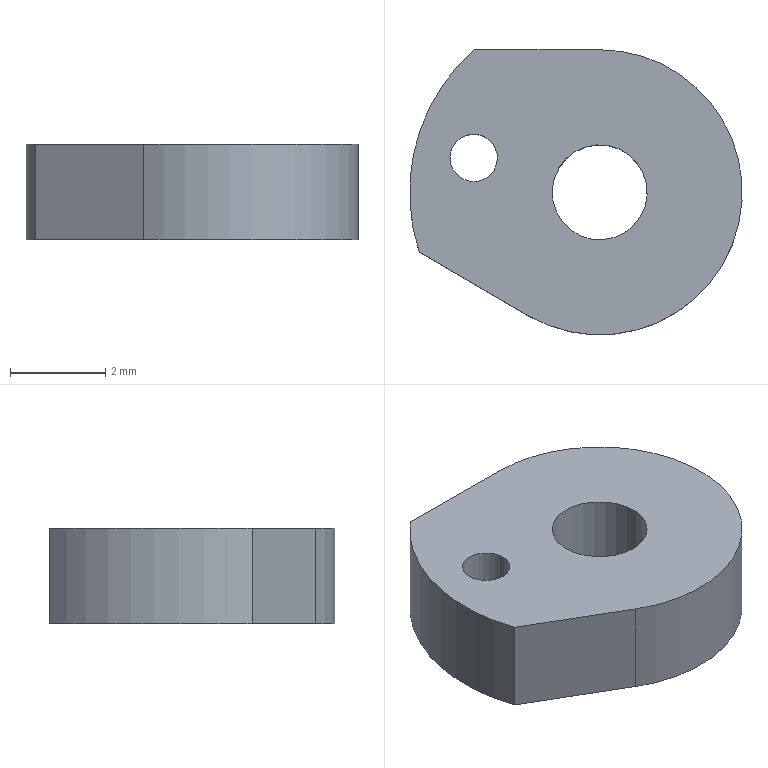Component | SolidWorks | DeflectionCam(Rear)-2 | 1 solid | 11 faces | box 7 x 6.01 x 2 mm | volume 60 mm3 | cylinder 7 | plane 4 | commonest cylinder face diameters 1 x2 2 x2 6 x2 8 x1
build123d program:
from build123d import *

# Parameters (mm, degrees)
SKETCH1_R           = 1
BOSS_EXTRUDE1_DEPTH = 2
SKETCH2_R           = 0.5
CUT_EXTRUDE1_DEPTH  = 2


with BuildPart() as part:
    # Sketch1 → Boss-Extrude1 (new body)
    with BuildSketch(Plane.XY):
        with BuildLine():
            Line((-5.155, 2.996), (-7.798, 2.859))
            ThreePointArc((-7.798, 2.859), (-8.912, 0.8339), (-8.72, -1.47))
            Line((-8.72, -1.47), (-6.363, -2.672))
            ThreePointArc((-6.363, -2.672), (-2.066, -0.6254), (-5.155, 2.996))
        make_face()
        with Locations((-5, 0)):
            Circle(SKETCH1_R, mode=Mode.SUBTRACT)
    extrude(amount=-BOSS_EXTRUDE1_DEPTH)

    # Sketch2 → Cut-Extrude1 (cut)
    with BuildSketch(Plane.XY):
        with Locations((-7.69, 0.5733)):
            Circle(SKETCH2_R)
    extrude(amount=-CUT_EXTRUDE1_DEPTH, mode=Mode.SUBTRACT)


solid = part.part

# Placed as in the assembly
solid = solid.moved(Location((17.492, -3.781, 7), (0, 0, -3.225)))
STEP:
#1=COLOUR_RGB('',0.7922,0.8196,0.9333);
#2=FILL_AREA_STYLE_COLOUR('',#1);
#3=FILL_AREA_STYLE('',(#2));
#4=SURFACE_STYLE_FILL_AREA(#3);
#5=SURFACE_SIDE_STYLE('',(#4));
#6=SURFACE_STYLE_USAGE(.BOTH.,#5);
#7=PRESENTATION_STYLE_ASSIGNMENT((#6));
#8=CARTESIAN_POINT('',(0.368,-0.1082,0.1969));
#9=VERTEX_POINT('',#8);
#10=CARTESIAN_POINT('',(0.4073,-0.1104,0.1969));
#11=VERTEX_POINT('',#10);
#12=CARTESIAN_POINT('',(0.3877,-0.1093,0.1969));
#13=DIRECTION('',(-0.,-0.,1.));
#14=DIRECTION('',(0.9984,-0.05626,0.));
#15=AXIS2_PLACEMENT_3D('',#12,#13,#14);
#16=CIRCLE('',#15,0.01969);
#17=EDGE_CURVE('',#9,#11,#16,.T.);
#18=ORIENTED_EDGE('',*,*,#17,.F.);
#19=CARTESIAN_POINT('',(0.368,-0.1082,0.2756));
#20=VERTEX_POINT('',#19);
#21=CARTESIAN_POINT('',(0.368,-0.1082,0.1969));
#22=DIRECTION('',(-0.,-0.,1.));
#23=VECTOR('',#22,39.37);
#24=LINE('',#21,#23);
#25=EDGE_CURVE('',#9,#20,#24,.T.);
#26=ORIENTED_EDGE('',*,*,#25,.T.);
#27=CARTESIAN_POINT('',(0.4073,-0.1104,0.2756));
#28=VERTEX_POINT('',#27);
#29=CARTESIAN_POINT('',(0.3877,-0.1093,0.2756));
#30=DIRECTION('',(-0.,-0.,1.));
#31=DIRECTION('',(0.9984,-0.05626,0.));
#32=AXIS2_PLACEMENT_3D('',#29,#30,#31);
#33=CIRCLE('',#32,0.01969);
#34=EDGE_CURVE('',#20,#28,#33,.T.);
#35=ORIENTED_EDGE('',*,*,#34,.T.);
#36=CARTESIAN_POINT('',(0.4073,-0.1104,0.1969));
#37=DIRECTION('',(-0.,-0.,1.));
#38=VECTOR('',#37,39.37);
#39=LINE('',#36,#38);
#40=EDGE_CURVE('',#11,#28,#39,.T.);
#41=ORIENTED_EDGE('',*,*,#40,.F.);
#42=EDGE_LOOP('',(#18,#26,#35,#41));
#43=FACE_OUTER_BOUND('',#42,.T.);
#44=CARTESIAN_POINT('',(0.3877,-0.1093,0.1969));
#45=DIRECTION('',(-0.,-0.,1.));
#46=DIRECTION('',(0.9984,-0.05626,0.));
#47=AXIS2_PLACEMENT_3D('',#44,#45,#46);
#48=CYLINDRICAL_SURFACE('',#47,0.01969);
#49=ADVANCED_FACE('',(#43),#48,.F.);
#50=CARTESIAN_POINT('',(0.4528,-0.1356,0.1969));
#51=VERTEX_POINT('',#50);
#52=CARTESIAN_POINT('',(0.5314,-0.14,0.1969));
#53=VERTEX_POINT('',#52);
#54=CARTESIAN_POINT('',(0.4921,-0.1378,0.1969));
#55=DIRECTION('',(-0.,-0.,1.));
#56=DIRECTION('',(0.9984,-0.05626,0.));
#57=AXIS2_PLACEMENT_3D('',#54,#55,#56);
#58=CIRCLE('',#57,0.03937);
#59=EDGE_CURVE('',#51,#53,#58,.T.);
#60=ORIENTED_EDGE('',*,*,#59,.F.);
#61=CARTESIAN_POINT('',(0.4528,-0.1356,0.2756));
#62=VERTEX_POINT('',#61);
#63=CARTESIAN_POINT('',(0.4528,-0.1356,0.1969));
#64=DIRECTION('',(-0.,-0.,1.));
#65=VECTOR('',#64,39.37);
#66=LINE('',#63,#65);
#67=EDGE_CURVE('',#51,#62,#66,.T.);
#68=ORIENTED_EDGE('',*,*,#67,.T.);
#69=CARTESIAN_POINT('',(0.5314,-0.14,0.2756));
#70=VERTEX_POINT('',#69);
#71=CARTESIAN_POINT('',(0.4921,-0.1378,0.2756));
#72=DIRECTION('',(-0.,-0.,1.));
#73=DIRECTION('',(0.9984,-0.05626,0.));
#74=AXIS2_PLACEMENT_3D('',#71,#72,#73);
#75=CIRCLE('',#74,0.03937);
#76=EDGE_CURVE('',#62,#70,#75,.T.);
#77=ORIENTED_EDGE('',*,*,#76,.T.);
#78=CARTESIAN_POINT('',(0.5314,-0.14,0.1969));
#79=DIRECTION('',(-0.,-0.,1.));
#80=VECTOR('',#79,39.37);
#81=LINE('',#78,#80);
#82=EDGE_CURVE('',#53,#70,#81,.T.);
#83=ORIENTED_EDGE('',*,*,#82,.F.);
#84=EDGE_LOOP('',(#60,#68,#77,#83));
#85=FACE_OUTER_BOUND('',#84,.T.);
#86=CARTESIAN_POINT('',(0.4921,-0.1378,0.1969));
#87=DIRECTION('',(-0.,-0.,1.));
#88=DIRECTION('',(0.9984,-0.05626,0.));
#89=AXIS2_PLACEMENT_3D('',#86,#87,#88);
#90=CYLINDRICAL_SURFACE('',#89,0.03937);
#91=ADVANCED_FACE('',(#85),#90,.F.);
#92=CARTESIAN_POINT('',(0.4326,-0.2398,0.1969));
#93=VERTEX_POINT('',#92);
#94=CARTESIAN_POINT('',(0.61,-0.1444,0.1969));
#95=VERTEX_POINT('',#94);
#96=CARTESIAN_POINT('',(0.4921,-0.1378,0.1969));
#97=DIRECTION('',(-0.,-0.,1.));
#98=DIRECTION('',(0.9984,-0.05626,0.));
#99=AXIS2_PLACEMENT_3D('',#96,#97,#98);
#100=CIRCLE('',#99,0.1181);
#101=EDGE_CURVE('',#93,#95,#100,.T.);
#102=ORIENTED_EDGE('',*,*,#101,.T.);
#103=CARTESIAN_POINT('',(0.61,-0.1444,0.2756));
#104=VERTEX_POINT('',#103);
#105=CARTESIAN_POINT('',(0.61,-0.1444,0.1969));
#106=DIRECTION('',(-0.,-0.,1.));
#107=VECTOR('',#106,39.37);
#108=LINE('',#105,#107);
#109=EDGE_CURVE('',#95,#104,#108,.T.);
#110=ORIENTED_EDGE('',*,*,#109,.T.);
#111=CARTESIAN_POINT('',(0.4326,-0.2398,0.2756));
#112=VERTEX_POINT('',#111);
#113=CARTESIAN_POINT('',(0.4921,-0.1378,0.2756));
#114=DIRECTION('',(-0.,-0.,1.));
#115=DIRECTION('',(0.9984,-0.05626,0.));
#116=AXIS2_PLACEMENT_3D('',#113,#114,#115);
#117=CIRCLE('',#116,0.1181);
#118=EDGE_CURVE('',#112,#104,#117,.T.);
#119=ORIENTED_EDGE('',*,*,#118,.F.);
#120=CARTESIAN_POINT('',(0.4326,-0.2398,0.1969));
#121=DIRECTION('',(-0.,-0.,1.));
#122=VECTOR('',#121,39.37);
#123=LINE('',#120,#122);
#124=EDGE_CURVE('',#93,#112,#123,.T.);
#125=ORIENTED_EDGE('',*,*,#124,.F.);
#126=EDGE_LOOP('',(#102,#110,#119,#125));
#127=FACE_OUTER_BOUND('',#126,.T.);
#128=CARTESIAN_POINT('',(0.4921,-0.1378,0.1969));
#129=DIRECTION('',(-0.,-0.,1.));
#130=DIRECTION('',(0.9984,-0.05626,0.));
#131=AXIS2_PLACEMENT_3D('',#128,#129,#130);
#132=CYLINDRICAL_SURFACE('',#131,0.1181);
#133=ADVANCED_FACE('',(#127),#132,.T.);
#134=ORIENTED_EDGE('',*,*,#109,.F.);
#135=CARTESIAN_POINT('',(0.4927,-0.01969,0.1969));
#136=VERTEX_POINT('',#135);
#137=CARTESIAN_POINT('',(0.4921,-0.1378,0.1969));
#138=DIRECTION('',(-0.,-0.,1.));
#139=DIRECTION('',(0.9984,-0.05626,0.));
#140=AXIS2_PLACEMENT_3D('',#137,#138,#139);
#141=CIRCLE('',#140,0.1181);
#142=EDGE_CURVE('',#95,#136,#141,.T.);
#143=ORIENTED_EDGE('',*,*,#142,.T.);
#144=CARTESIAN_POINT('',(0.4927,-0.01969,0.2756));
#145=VERTEX_POINT('',#144);
#146=CARTESIAN_POINT('',(0.4927,-0.01969,0.1969));
#147=DIRECTION('',(-0.,-0.,1.));
#148=VECTOR('',#147,39.37);
#149=LINE('',#146,#148);
#150=EDGE_CURVE('',#136,#145,#149,.T.);
#151=ORIENTED_EDGE('',*,*,#150,.T.);
#152=CARTESIAN_POINT('',(0.4921,-0.1378,0.2756));
#153=DIRECTION('',(-0.,-0.,1.));
#154=DIRECTION('',(0.9984,-0.05626,0.));
#155=AXIS2_PLACEMENT_3D('',#152,#153,#154);
#156=CIRCLE('',#155,0.1181);
#157=EDGE_CURVE('',#104,#145,#156,.T.);
#158=ORIENTED_EDGE('',*,*,#157,.F.);
#159=EDGE_LOOP('',(#134,#143,#151,#158));
#160=FACE_OUTER_BOUND('',#159,.T.);
#161=CARTESIAN_POINT('',(0.4921,-0.1378,0.1969));
#162=DIRECTION('',(-0.,-0.,1.));
#163=DIRECTION('',(0.9984,-0.05626,0.));
#164=AXIS2_PLACEMENT_3D('',#161,#162,#163);
#165=CYLINDRICAL_SURFACE('',#164,0.1181);
#166=ADVANCED_FACE('',(#160),#165,.T.);
#167=CARTESIAN_POINT('',(0.3426,-0.1873,0.2756));
#168=VERTEX_POINT('',#167);
#169=CARTESIAN_POINT('',(0.4326,-0.2398,0.2756));
#170=DIRECTION('',(0.8638,-0.5039,0.));
#171=VECTOR('',#170,39.37);
#172=LINE('',#169,#171);
#173=EDGE_CURVE('',#168,#112,#172,.T.);
#174=ORIENTED_EDGE('',*,*,#173,.F.);
#175=CARTESIAN_POINT('',(0.3426,-0.1873,0.1969));
#176=VERTEX_POINT('',#175);
#177=CARTESIAN_POINT('',(0.3426,-0.1873,0.1969));
#178=DIRECTION('',(-0.,-0.,1.));
#179=VECTOR('',#178,39.37);
#180=LINE('',#177,#179);
#181=EDGE_CURVE('',#176,#168,#180,.T.);
#182=ORIENTED_EDGE('',*,*,#181,.F.);
#183=CARTESIAN_POINT('',(0.4326,-0.2398,0.1969));
#184=DIRECTION('',(0.8638,-0.5039,0.));
#185=VECTOR('',#184,39.37);
#186=LINE('',#183,#185);
#187=EDGE_CURVE('',#176,#93,#186,.T.);
#188=ORIENTED_EDGE('',*,*,#187,.T.);
#189=ORIENTED_EDGE('',*,*,#124,.T.);
#190=EDGE_LOOP('',(#174,#182,#188,#189));
#191=FACE_OUTER_BOUND('',#190,.T.);
#192=CARTESIAN_POINT('',(0.4326,-0.2398,0.1969));
#193=DIRECTION('',(-0.5039,-0.8638,0.));
#194=DIRECTION('',(0.8638,-0.5039,0.));
#195=AXIS2_PLACEMENT_3D('',#192,#193,#194);
#196=PLANE('',#195);
#197=ADVANCED_FACE('',(#191),#196,.T.);
#198=CARTESIAN_POINT('',(0.3885,-0.01922,0.2756));
#199=VERTEX_POINT('',#198);
#200=CARTESIAN_POINT('',(0.4921,-0.1378,0.2756));
#201=DIRECTION('',(-0.,-0.,1.));
#202=DIRECTION('',(0.9984,-0.05626,0.));
#203=AXIS2_PLACEMENT_3D('',#200,#201,#202);
#204=CIRCLE('',#203,0.1575);
#205=EDGE_CURVE('',#199,#168,#204,.T.);
#206=ORIENTED_EDGE('',*,*,#205,.F.);
#207=CARTESIAN_POINT('',(0.3885,-0.01922,0.1969));
#208=VERTEX_POINT('',#207);
#209=CARTESIAN_POINT('',(0.3885,-0.01922,0.1969));
#210=DIRECTION('',(-0.,-0.,1.));
#211=VECTOR('',#210,39.37);
#212=LINE('',#209,#211);
#213=EDGE_CURVE('',#208,#199,#212,.T.);
#214=ORIENTED_EDGE('',*,*,#213,.F.);
#215=CARTESIAN_POINT('',(0.4921,-0.1378,0.1969));
#216=DIRECTION('',(-0.,-0.,1.));
#217=DIRECTION('',(0.9984,-0.05626,0.));
#218=AXIS2_PLACEMENT_3D('',#215,#216,#217);
#219=CIRCLE('',#218,0.1575);
#220=EDGE_CURVE('',#208,#176,#219,.T.);
#221=ORIENTED_EDGE('',*,*,#220,.T.);
#222=ORIENTED_EDGE('',*,*,#181,.T.);
#223=EDGE_LOOP('',(#206,#214,#221,#222));
#224=FACE_OUTER_BOUND('',#223,.T.);
#225=CARTESIAN_POINT('',(0.4921,-0.1378,0.1969));
#226=DIRECTION('',(-0.,-0.,1.));
#227=DIRECTION('',(0.9984,-0.05626,0.));
#228=AXIS2_PLACEMENT_3D('',#225,#226,#227);
#229=CYLINDRICAL_SURFACE('',#228,0.1575);
#230=ADVANCED_FACE('',(#224),#229,.T.);
#231=CARTESIAN_POINT('',(0.4927,-0.01969,0.2756));
#232=DIRECTION('',(-1.,0.004495,0.));
#233=VECTOR('',#232,39.37);
#234=LINE('',#231,#233);
#235=EDGE_CURVE('',#145,#199,#234,.T.);
#236=ORIENTED_EDGE('',*,*,#235,.F.);
#237=ORIENTED_EDGE('',*,*,#150,.F.);
#238=CARTESIAN_POINT('',(0.4927,-0.01969,0.1969));
#239=DIRECTION('',(-1.,0.004495,0.));
#240=VECTOR('',#239,39.37);
#241=LINE('',#238,#240);
#242=EDGE_CURVE('',#136,#208,#241,.T.);
#243=ORIENTED_EDGE('',*,*,#242,.T.);
#244=ORIENTED_EDGE('',*,*,#213,.T.);
#245=EDGE_LOOP('',(#236,#237,#243,#244));
#246=FACE_OUTER_BOUND('',#245,.T.);
#247=CARTESIAN_POINT('',(0.4927,-0.01969,0.1969));
#248=DIRECTION('',(0.004495,1.,-0.));
#249=DIRECTION('',(-1.,0.004495,0.));
#250=AXIS2_PLACEMENT_3D('',#247,#248,#249);
#251=PLANE('',#250);
#252=ADVANCED_FACE('',(#246),#251,.T.);
#253=CARTESIAN_POINT('',(0.3877,-0.1093,0.1969));
#254=DIRECTION('',(-0.,-0.,1.));
#255=DIRECTION('',(0.9984,-0.05626,0.));
#256=AXIS2_PLACEMENT_3D('',#253,#254,#255);
#257=CIRCLE('',#256,0.01969);
#258=EDGE_CURVE('',#11,#9,#257,.T.);
#259=ORIENTED_EDGE('',*,*,#258,.T.);
#260=ORIENTED_EDGE('',*,*,#17,.T.);
#261=EDGE_LOOP('',(#259,#260));
#262=FACE_BOUND('',#261,.T.);
#263=CARTESIAN_POINT('',(0.4921,-0.1378,0.1969));
#264=DIRECTION('',(-0.,-0.,1.));
#265=DIRECTION('',(0.9984,-0.05626,0.));
#266=AXIS2_PLACEMENT_3D('',#263,#264,#265);
#267=CIRCLE('',#266,0.03937);
#268=EDGE_CURVE('',#53,#51,#267,.T.);
#269=ORIENTED_EDGE('',*,*,#268,.T.);
#270=ORIENTED_EDGE('',*,*,#59,.T.);
#271=EDGE_LOOP('',(#269,#270));
#272=FACE_BOUND('',#271,.T.);
#273=ORIENTED_EDGE('',*,*,#101,.F.);
#274=ORIENTED_EDGE('',*,*,#187,.F.);
#275=ORIENTED_EDGE('',*,*,#220,.F.);
#276=ORIENTED_EDGE('',*,*,#242,.F.);
#277=ORIENTED_EDGE('',*,*,#142,.F.);
#278=EDGE_LOOP('',(#273,#274,#275,#276,#277));
#279=FACE_OUTER_BOUND('',#278,.T.);
#280=CARTESIAN_POINT('',(0.4921,-0.1378,0.1969));
#281=DIRECTION('',(0.,-0.,1.));
#282=DIRECTION('',(0.9984,-0.05626,-0.));
#283=AXIS2_PLACEMENT_3D('',#280,#281,#282);
#284=PLANE('',#283);
#285=ADVANCED_FACE('',(#262,#272,#279),#284,.F.);
#286=CARTESIAN_POINT('',(0.3877,-0.1093,0.2756));
#287=DIRECTION('',(-0.,-0.,1.));
#288=DIRECTION('',(0.9984,-0.05626,0.));
#289=AXIS2_PLACEMENT_3D('',#286,#287,#288);
#290=CIRCLE('',#289,0.01969);
#291=EDGE_CURVE('',#28,#20,#290,.T.);
#292=ORIENTED_EDGE('',*,*,#291,.F.);
#293=ORIENTED_EDGE('',*,*,#34,.F.);
#294=EDGE_LOOP('',(#292,#293));
#295=FACE_BOUND('',#294,.T.);
#296=CARTESIAN_POINT('',(0.4921,-0.1378,0.2756));
#297=DIRECTION('',(-0.,-0.,1.));
#298=DIRECTION('',(0.9984,-0.05626,0.));
#299=AXIS2_PLACEMENT_3D('',#296,#297,#298);
#300=CIRCLE('',#299,0.03937);
#301=EDGE_CURVE('',#70,#62,#300,.T.);
#302=ORIENTED_EDGE('',*,*,#301,.F.);
#303=ORIENTED_EDGE('',*,*,#76,.F.);
#304=EDGE_LOOP('',(#302,#303));
#305=FACE_BOUND('',#304,.T.);
#306=ORIENTED_EDGE('',*,*,#118,.T.);
#307=ORIENTED_EDGE('',*,*,#157,.T.);
#308=ORIENTED_EDGE('',*,*,#235,.T.);
#309=ORIENTED_EDGE('',*,*,#205,.T.);
#310=ORIENTED_EDGE('',*,*,#173,.T.);
#311=EDGE_LOOP('',(#306,#307,#308,#309,#310));
#312=FACE_OUTER_BOUND('',#311,.T.);
#313=CARTESIAN_POINT('',(0.4921,-0.1378,0.2756));
#314=DIRECTION('',(0.,-0.,1.));
#315=DIRECTION('',(0.9984,-0.05626,-0.));
#316=AXIS2_PLACEMENT_3D('',#313,#314,#315);
#317=PLANE('',#316);
#318=ADVANCED_FACE('',(#295,#305,#312),#317,.T.);
#319=ORIENTED_EDGE('',*,*,#67,.F.);
#320=ORIENTED_EDGE('',*,*,#268,.F.);
#321=ORIENTED_EDGE('',*,*,#82,.T.);
#322=ORIENTED_EDGE('',*,*,#301,.T.);
#323=EDGE_LOOP('',(#319,#320,#321,#322));
#324=FACE_OUTER_BOUND('',#323,.T.);
#325=CARTESIAN_POINT('',(0.4921,-0.1378,0.1969));
#326=DIRECTION('',(-0.,-0.,1.));
#327=DIRECTION('',(0.9984,-0.05626,0.));
#328=AXIS2_PLACEMENT_3D('',#325,#326,#327);
#329=CYLINDRICAL_SURFACE('',#328,0.03937);
#330=ADVANCED_FACE('',(#324),#329,.F.);
#331=ORIENTED_EDGE('',*,*,#25,.F.);
#332=ORIENTED_EDGE('',*,*,#258,.F.);
#333=ORIENTED_EDGE('',*,*,#40,.T.);
#334=ORIENTED_EDGE('',*,*,#291,.T.);
#335=EDGE_LOOP('',(#331,#332,#333,#334));
#336=FACE_OUTER_BOUND('',#335,.T.);
#337=CARTESIAN_POINT('',(0.3877,-0.1093,0.1969));
#338=DIRECTION('',(-0.,-0.,1.));
#339=DIRECTION('',(0.9984,-0.05626,0.));
#340=AXIS2_PLACEMENT_3D('',#337,#338,#339);
#341=CYLINDRICAL_SURFACE('',#340,0.01969);
#342=ADVANCED_FACE('',(#336),#341,.F.);
#343=CLOSED_SHELL('',(#49,#91,#133,#166,#197,#230,#252,#285,#318,#330,#342));
#344=MANIFOLD_SOLID_BREP('',#343);
#345=STYLED_ITEM('',(#7),#344);
#346=(LENGTH_UNIT()NAMED_UNIT(*)SI_UNIT($,.METRE.));
#347=LENGTH_MEASURE_WITH_UNIT(LENGTH_MEASURE(0.0254),#346);
#348=DIMENSIONAL_EXPONENTS(1.,0.,0.,0.,0.,0.,0.);
#349=(CONVERSION_BASED_UNIT('',#347)LENGTH_UNIT()NAMED_UNIT(#348));
#350=UNCERTAINTY_MEASURE_WITH_UNIT(LENGTH_MEASURE(0.00001),#349,'','');
#351=(NAMED_UNIT(*)PLANE_ANGLE_UNIT()SI_UNIT($,.RADIAN.));
#352=(NAMED_UNIT(*)SI_UNIT($,.STERADIAN.)SOLID_ANGLE_UNIT());
#353=(GEOMETRIC_REPRESENTATION_CONTEXT(3)GLOBAL_UNCERTAINTY_ASSIGNED_CONTEXT((#350))GLOBAL_UNIT_ASSIGNED_CONTEXT((#349,#351,#352))REPRESENTATION_CONTEXT('',''));
#354=MECHANICAL_DESIGN_GEOMETRIC_PRESENTATION_REPRESENTATION('',(#345),#353);
#355=CARTESIAN_POINT('',(0.,0.,0.));
#356=DIRECTION('',(0.,0.,1.));
#357=DIRECTION('',(1.,0.,0.));
#358=AXIS2_PLACEMENT_3D('',#355,#356,#357);
#359=(LENGTH_UNIT()NAMED_UNIT(*)SI_UNIT($,.METRE.));
#360=LENGTH_MEASURE_WITH_UNIT(LENGTH_MEASURE(0.0254),#359);
#361=DIMENSIONAL_EXPONENTS(1.,0.,0.,0.,0.,0.,0.);
#362=(CONVERSION_BASED_UNIT('',#360)LENGTH_UNIT()NAMED_UNIT(#361));
#363=UNCERTAINTY_MEASURE_WITH_UNIT(LENGTH_MEASURE(0.00001),#362,'','');
#364=(NAMED_UNIT(*)PLANE_ANGLE_UNIT()SI_UNIT($,.RADIAN.));
#365=(NAMED_UNIT(*)SI_UNIT($,.STERADIAN.)SOLID_ANGLE_UNIT());
#366=(GEOMETRIC_REPRESENTATION_CONTEXT(3)GLOBAL_UNCERTAINTY_ASSIGNED_CONTEXT((#363))GLOBAL_UNIT_ASSIGNED_CONTEXT((#362,#364,#365))REPRESENTATION_CONTEXT('',''));
#367=ADVANCED_BREP_SHAPE_REPRESENTATION('',(#344,#358),#366);
#368=PRESENTATION_LAYER_ASSIGNMENT('','',(#345));